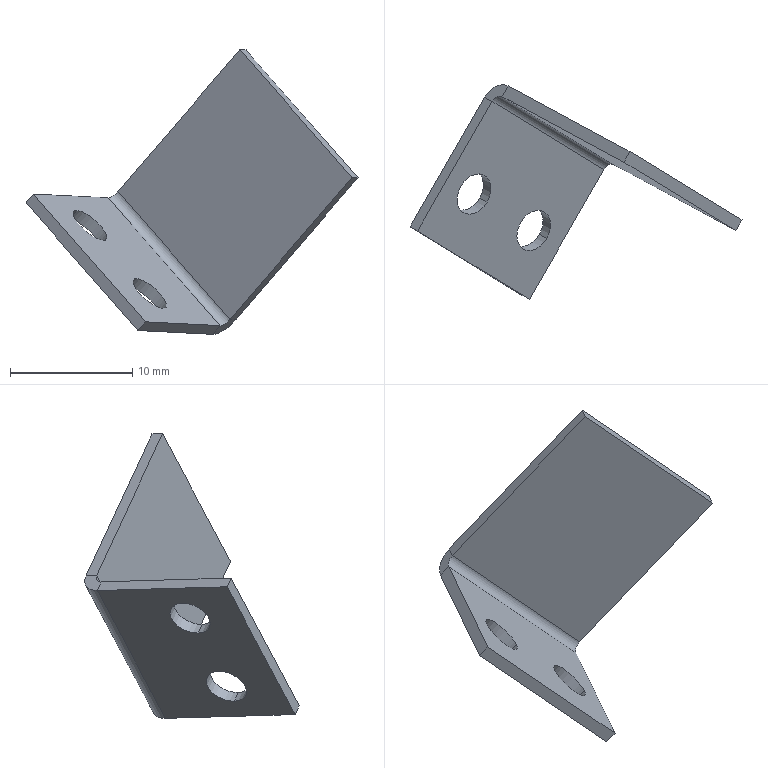Component | SolidWorks | ShadingPlateZ0-123-1 | 1 solid | 18 faces | box 27.21 x 17.57 x 23.33 mm | volume 438 mm3 | plane 12 | cylinder 6 | commonest cylinder face diameters 3.5 x4 3.473 x1 1.473 x1
STEP:
#1=COLOUR_RGB('',0.7922,0.8196,0.9333);
#2=FILL_AREA_STYLE_COLOUR('',#1);
#3=FILL_AREA_STYLE('',(#2));
#4=SURFACE_STYLE_FILL_AREA(#3);
#5=SURFACE_SIDE_STYLE('',(#4));
#6=SURFACE_STYLE_USAGE(.BOTH.,#5);
#7=PRESENTATION_STYLE_ASSIGNMENT((#6));
#8=CARTESIAN_POINT('',(2.839,-1.342,7.329));
#9=VERTEX_POINT('',#8);
#10=CARTESIAN_POINT('',(2.755,-1.29,7.425));
#11=VERTEX_POINT('',#10);
#12=CARTESIAN_POINT('',(2.797,-1.316,7.377));
#13=DIRECTION('',(0.6147,-0.3321,0.7154));
#14=DIRECTION('',(-0.6119,0.3716,0.6982));
#15=AXIS2_PLACEMENT_3D('',#12,#13,#14);
#16=CIRCLE('',#15,0.0689);
#17=EDGE_CURVE('',#9,#11,#16,.T.);
#18=ORIENTED_EDGE('',*,*,#17,.F.);
#19=CARTESIAN_POINT('',(2.864,-1.355,7.357));
#20=VERTEX_POINT('',#19);
#21=CARTESIAN_POINT('',(2.839,-1.342,7.329));
#22=DIRECTION('',(0.6147,-0.3321,0.7154));
#23=VECTOR('',#22,39.37);
#24=LINE('',#21,#23);
#25=EDGE_CURVE('',#9,#20,#24,.T.);
#26=ORIENTED_EDGE('',*,*,#25,.T.);
#27=CARTESIAN_POINT('',(2.779,-1.304,7.453));
#28=VERTEX_POINT('',#27);
#29=CARTESIAN_POINT('',(2.821,-1.329,7.405));
#30=DIRECTION('',(0.6147,-0.3321,0.7154));
#31=DIRECTION('',(-0.6119,0.3716,0.6982));
#32=AXIS2_PLACEMENT_3D('',#29,#30,#31);
#33=CIRCLE('',#32,0.0689);
#34=EDGE_CURVE('',#20,#28,#33,.T.);
#35=ORIENTED_EDGE('',*,*,#34,.T.);
#36=CARTESIAN_POINT('',(2.755,-1.29,7.425));
#37=DIRECTION('',(0.6147,-0.3321,0.7154));
#38=VECTOR('',#37,39.37);
#39=LINE('',#36,#38);
#40=EDGE_CURVE('',#11,#28,#39,.T.);
#41=ORIENTED_EDGE('',*,*,#40,.F.);
#42=EDGE_LOOP('',(#18,#26,#35,#41));
#43=FACE_OUTER_BOUND('',#42,.T.);
#44=CARTESIAN_POINT('',(2.797,-1.316,7.377));
#45=DIRECTION('',(0.6147,-0.3321,0.7154));
#46=DIRECTION('',(-0.6119,0.3716,0.6982));
#47=AXIS2_PLACEMENT_3D('',#44,#45,#46);
#48=CYLINDRICAL_SURFACE('',#47,0.0689);
#49=ADVANCED_FACE('',(#43),#48,.F.);
#50=CARTESIAN_POINT('',(3.032,-1.459,7.109));
#51=VERTEX_POINT('',#50);
#52=CARTESIAN_POINT('',(2.948,-1.407,7.205));
#53=VERTEX_POINT('',#52);
#54=CARTESIAN_POINT('',(2.99,-1.433,7.157));
#55=DIRECTION('',(0.6147,-0.3321,0.7154));
#56=DIRECTION('',(-0.6119,0.3716,0.6982));
#57=AXIS2_PLACEMENT_3D('',#54,#55,#56);
#58=CIRCLE('',#57,0.0689);
#59=EDGE_CURVE('',#51,#53,#58,.T.);
#60=ORIENTED_EDGE('',*,*,#59,.F.);
#61=CARTESIAN_POINT('',(3.056,-1.472,7.137));
#62=VERTEX_POINT('',#61);
#63=CARTESIAN_POINT('',(3.032,-1.459,7.109));
#64=DIRECTION('',(0.6147,-0.3321,0.7154));
#65=VECTOR('',#64,39.37);
#66=LINE('',#63,#65);
#67=EDGE_CURVE('',#51,#62,#66,.T.);
#68=ORIENTED_EDGE('',*,*,#67,.T.);
#69=CARTESIAN_POINT('',(2.972,-1.421,7.233));
#70=VERTEX_POINT('',#69);
#71=CARTESIAN_POINT('',(3.014,-1.446,7.185));
#72=DIRECTION('',(0.6147,-0.3321,0.7154));
#73=DIRECTION('',(-0.6119,0.3716,0.6982));
#74=AXIS2_PLACEMENT_3D('',#71,#72,#73);
#75=CIRCLE('',#74,0.0689);
#76=EDGE_CURVE('',#62,#70,#75,.T.);
#77=ORIENTED_EDGE('',*,*,#76,.T.);
#78=CARTESIAN_POINT('',(2.948,-1.407,7.205));
#79=DIRECTION('',(0.6147,-0.3321,0.7154));
#80=VECTOR('',#79,39.37);
#81=LINE('',#78,#80);
#82=EDGE_CURVE('',#53,#70,#81,.T.);
#83=ORIENTED_EDGE('',*,*,#82,.F.);
#84=EDGE_LOOP('',(#60,#68,#77,#83));
#85=FACE_OUTER_BOUND('',#84,.T.);
#86=CARTESIAN_POINT('',(2.99,-1.433,7.157));
#87=DIRECTION('',(0.6147,-0.3321,0.7154));
#88=DIRECTION('',(-0.6119,0.3716,0.6982));
#89=AXIS2_PLACEMENT_3D('',#86,#87,#88);
#90=CYLINDRICAL_SURFACE('',#89,0.0689);
#91=ADVANCED_FACE('',(#85),#90,.F.);
#92=CARTESIAN_POINT('',(2.879,-1.03,7.494));
#93=VERTEX_POINT('',#92);
#94=CARTESIAN_POINT('',(2.639,-1.449,7.506));
#95=VERTEX_POINT('',#94);
#96=CARTESIAN_POINT('',(2.639,-1.449,7.506));
#97=DIRECTION('',(-0.4977,-0.867,0.02519));
#98=VECTOR('',#97,39.37);
#99=LINE('',#96,#98);
#100=EDGE_CURVE('',#93,#95,#99,.T.);
#101=ORIENTED_EDGE('',*,*,#100,.F.);
#102=CARTESIAN_POINT('',(2.855,-1.017,7.466));
#103=VERTEX_POINT('',#102);
#104=CARTESIAN_POINT('',(2.879,-1.03,7.494));
#105=DIRECTION('',(-0.6147,0.3321,-0.7154));
#106=VECTOR('',#105,39.37);
#107=LINE('',#104,#106);
#108=EDGE_CURVE('',#93,#103,#107,.T.);
#109=ORIENTED_EDGE('',*,*,#108,.T.);
#110=CARTESIAN_POINT('',(2.615,-1.435,7.478));
#111=VERTEX_POINT('',#110);
#112=CARTESIAN_POINT('',(2.615,-1.435,7.478));
#113=DIRECTION('',(-0.4977,-0.867,0.02519));
#114=VECTOR('',#113,39.37);
#115=LINE('',#112,#114);
#116=EDGE_CURVE('',#103,#111,#115,.T.);
#117=ORIENTED_EDGE('',*,*,#116,.T.);
#118=CARTESIAN_POINT('',(2.615,-1.435,7.478));
#119=DIRECTION('',(0.6147,-0.3321,0.7154));
#120=VECTOR('',#119,39.37);
#121=LINE('',#118,#120);
#122=EDGE_CURVE('',#111,#95,#121,.T.);
#123=ORIENTED_EDGE('',*,*,#122,.T.);
#124=EDGE_LOOP('',(#101,#109,#117,#123));
#125=FACE_OUTER_BOUND('',#124,.T.);
#126=CARTESIAN_POINT('',(2.615,-1.435,7.478));
#127=DIRECTION('',(-0.6119,0.3716,0.6982));
#128=DIRECTION('',(-0.4977,-0.867,0.02519));
#129=AXIS2_PLACEMENT_3D('',#126,#127,#128);
#130=PLANE('',#129);
#131=ADVANCED_FACE('',(#125),#130,.T.);
#132=CARTESIAN_POINT('',(2.797,-1.316,7.377));
#133=DIRECTION('',(0.6147,-0.3321,0.7154));
#134=DIRECTION('',(-0.6119,0.3716,0.6982));
#135=AXIS2_PLACEMENT_3D('',#132,#133,#134);
#136=CIRCLE('',#135,0.0689);
#137=EDGE_CURVE('',#11,#9,#136,.T.);
#138=ORIENTED_EDGE('',*,*,#137,.T.);
#139=ORIENTED_EDGE('',*,*,#17,.T.);
#140=EDGE_LOOP('',(#138,#139));
#141=FACE_BOUND('',#140,.T.);
#142=CARTESIAN_POINT('',(2.99,-1.433,7.157));
#143=DIRECTION('',(0.6147,-0.3321,0.7154));
#144=DIRECTION('',(-0.6119,0.3716,0.6982));
#145=AXIS2_PLACEMENT_3D('',#142,#143,#144);
#146=CIRCLE('',#145,0.0689);
#147=EDGE_CURVE('',#53,#51,#146,.T.);
#148=ORIENTED_EDGE('',*,*,#147,.T.);
#149=ORIENTED_EDGE('',*,*,#59,.T.);
#150=EDGE_LOOP('',(#148,#149));
#151=FACE_BOUND('',#150,.T.);
#152=CARTESIAN_POINT('',(3.217,-1.236,7.054));
#153=VERTEX_POINT('',#152);
#154=CARTESIAN_POINT('',(2.855,-1.017,7.466));
#155=DIRECTION('',(0.6119,-0.3716,-0.6982));
#156=VECTOR('',#155,39.37);
#157=LINE('',#154,#156);
#158=EDGE_CURVE('',#103,#153,#157,.T.);
#159=ORIENTED_EDGE('',*,*,#158,.T.);
#160=CARTESIAN_POINT('',(2.976,-1.655,7.066));
#161=VERTEX_POINT('',#160);
#162=CARTESIAN_POINT('',(2.976,-1.655,7.066));
#163=DIRECTION('',(0.4977,0.867,-0.02519));
#164=VECTOR('',#163,39.37);
#165=LINE('',#162,#164);
#166=EDGE_CURVE('',#161,#153,#165,.T.);
#167=ORIENTED_EDGE('',*,*,#166,.F.);
#168=CARTESIAN_POINT('',(2.976,-1.655,7.066));
#169=DIRECTION('',(0.6119,-0.3716,-0.6982));
#170=VECTOR('',#169,39.37);
#171=LINE('',#168,#170);
#172=EDGE_CURVE('',#111,#161,#171,.T.);
#173=ORIENTED_EDGE('',*,*,#172,.F.);
#174=ORIENTED_EDGE('',*,*,#116,.F.);
#175=EDGE_LOOP('',(#159,#167,#173,#174));
#176=FACE_OUTER_BOUND('',#175,.T.);
#177=CARTESIAN_POINT('',(2.923,-1.323,7.265));
#178=DIRECTION('',(0.6147,-0.3321,0.7154));
#179=DIRECTION('',(-0.6119,0.3716,0.6982));
#180=AXIS2_PLACEMENT_3D('',#177,#178,#179);
#181=PLANE('',#180);
#182=ADVANCED_FACE('',(#141,#151,#176),#181,.F.);
#183=CARTESIAN_POINT('',(2.821,-1.329,7.405));
#184=DIRECTION('',(0.6147,-0.3321,0.7154));
#185=DIRECTION('',(-0.6119,0.3716,0.6982));
#186=AXIS2_PLACEMENT_3D('',#183,#184,#185);
#187=CIRCLE('',#186,0.0689);
#188=EDGE_CURVE('',#28,#20,#187,.T.);
#189=ORIENTED_EDGE('',*,*,#188,.F.);
#190=ORIENTED_EDGE('',*,*,#34,.F.);
#191=EDGE_LOOP('',(#189,#190));
#192=FACE_BOUND('',#191,.T.);
#193=CARTESIAN_POINT('',(3.014,-1.446,7.185));
#194=DIRECTION('',(0.6147,-0.3321,0.7154));
#195=DIRECTION('',(-0.6119,0.3716,0.6982));
#196=AXIS2_PLACEMENT_3D('',#193,#194,#195);
#197=CIRCLE('',#196,0.0689);
#198=EDGE_CURVE('',#70,#62,#197,.T.);
#199=ORIENTED_EDGE('',*,*,#198,.F.);
#200=ORIENTED_EDGE('',*,*,#76,.F.);
#201=EDGE_LOOP('',(#199,#200));
#202=FACE_BOUND('',#201,.T.);
#203=CARTESIAN_POINT('',(3.,-1.668,7.094));
#204=VERTEX_POINT('',#203);
#205=CARTESIAN_POINT('',(3.241,-1.249,7.082));
#206=VERTEX_POINT('',#205);
#207=CARTESIAN_POINT('',(3.,-1.668,7.094));
#208=DIRECTION('',(0.4977,0.867,-0.02519));
#209=VECTOR('',#208,39.37);
#210=LINE('',#207,#209);
#211=EDGE_CURVE('',#204,#206,#210,.T.);
#212=ORIENTED_EDGE('',*,*,#211,.T.);
#213=CARTESIAN_POINT('',(2.879,-1.03,7.494));
#214=DIRECTION('',(0.6119,-0.3716,-0.6982));
#215=VECTOR('',#214,39.37);
#216=LINE('',#213,#215);
#217=EDGE_CURVE('',#93,#206,#216,.T.);
#218=ORIENTED_EDGE('',*,*,#217,.F.);
#219=ORIENTED_EDGE('',*,*,#100,.T.);
#220=CARTESIAN_POINT('',(3.,-1.668,7.094));
#221=DIRECTION('',(0.6119,-0.3716,-0.6982));
#222=VECTOR('',#221,39.37);
#223=LINE('',#220,#222);
#224=EDGE_CURVE('',#95,#204,#223,.T.);
#225=ORIENTED_EDGE('',*,*,#224,.T.);
#226=EDGE_LOOP('',(#212,#218,#219,#225));
#227=FACE_OUTER_BOUND('',#226,.T.);
#228=CARTESIAN_POINT('',(2.947,-1.336,7.294));
#229=DIRECTION('',(0.6147,-0.3321,0.7154));
#230=DIRECTION('',(-0.6119,0.3716,0.6982));
#231=AXIS2_PLACEMENT_3D('',#228,#229,#230);
#232=PLANE('',#231);
#233=ADVANCED_FACE('',(#192,#202,#227),#232,.T.);
#234=CARTESIAN_POINT('',(3.241,-1.249,7.082));
#235=DIRECTION('',(-0.6147,0.3321,-0.7154));
#236=VECTOR('',#235,39.37);
#237=LINE('',#234,#236);
#238=EDGE_CURVE('',#206,#153,#237,.T.);
#239=ORIENTED_EDGE('',*,*,#238,.F.);
#240=ORIENTED_EDGE('',*,*,#211,.F.);
#241=CARTESIAN_POINT('',(2.976,-1.655,7.066));
#242=DIRECTION('',(0.6147,-0.3321,0.7154));
#243=VECTOR('',#242,39.37);
#244=LINE('',#241,#243);
#245=EDGE_CURVE('',#161,#204,#244,.T.);
#246=ORIENTED_EDGE('',*,*,#245,.F.);
#247=ORIENTED_EDGE('',*,*,#166,.T.);
#248=EDGE_LOOP('',(#239,#240,#246,#247));
#249=FACE_OUTER_BOUND('',#248,.T.);
#250=CARTESIAN_POINT('',(2.976,-1.655,7.066));
#251=DIRECTION('',(0.6119,-0.3716,-0.6982));
#252=DIRECTION('',(0.4977,0.867,-0.02519));
#253=AXIS2_PLACEMENT_3D('',#250,#251,#252);
#254=PLANE('',#253);
#255=ADVANCED_FACE('',(#249),#254,.T.);
#256=ORIENTED_EDGE('',*,*,#224,.F.);
#257=ORIENTED_EDGE('',*,*,#122,.F.);
#258=ORIENTED_EDGE('',*,*,#172,.T.);
#259=ORIENTED_EDGE('',*,*,#245,.T.);
#260=EDGE_LOOP('',(#256,#257,#258,#259));
#261=FACE_OUTER_BOUND('',#260,.T.);
#262=CARTESIAN_POINT('',(2.976,-1.655,7.066));
#263=DIRECTION('',(-0.4977,-0.867,0.02519));
#264=DIRECTION('',(0.6147,-0.3321,0.7154));
#265=AXIS2_PLACEMENT_3D('',#262,#263,#264);
#266=PLANE('',#265);
#267=ADVANCED_FACE('',(#261),#266,.T.);
#268=CARTESIAN_POINT('',(3.273,-1.234,7.102));
#269=VERTEX_POINT('',#268);
#270=CARTESIAN_POINT('',(3.293,-1.2,7.101));
#271=VERTEX_POINT('',#270);
#272=CARTESIAN_POINT('',(3.273,-1.234,7.102));
#273=DIRECTION('',(0.4977,0.867,-0.02519));
#274=VECTOR('',#273,39.37);
#275=LINE('',#272,#274);
#276=EDGE_CURVE('',#269,#271,#275,.T.);
#277=ORIENTED_EDGE('',*,*,#276,.F.);
#278=CARTESIAN_POINT('',(3.259,-1.259,7.102));
#279=DIRECTION('',(0.6119,-0.3716,-0.6982));
#280=DIRECTION('',(-0.6147,0.3321,-0.7154));
#281=AXIS2_PLACEMENT_3D('',#278,#279,#280);
#282=CIRCLE('',#281,0.029);
#283=EDGE_CURVE('',#206,#269,#282,.T.);
#284=ORIENTED_EDGE('',*,*,#283,.F.);
#285=ORIENTED_EDGE('',*,*,#238,.T.);
#286=CARTESIAN_POINT('',(3.259,-1.259,7.102));
#287=DIRECTION('',(0.6119,-0.3716,-0.6982));
#288=DIRECTION('',(-0.6147,0.3321,-0.7154));
#289=AXIS2_PLACEMENT_3D('',#286,#287,#288);
#290=CIRCLE('',#289,0.06837);
#291=EDGE_CURVE('',#153,#271,#290,.T.);
#292=ORIENTED_EDGE('',*,*,#291,.T.);
#293=EDGE_LOOP('',(#277,#284,#285,#292));
#294=FACE_OUTER_BOUND('',#293,.T.);
#295=CARTESIAN_POINT('',(3.259,-1.259,7.102));
#296=DIRECTION('',(0.6119,-0.3716,-0.6982));
#297=DIRECTION('',(0.6147,-0.3321,0.7154));
#298=AXIS2_PLACEMENT_3D('',#295,#296,#297);
#299=PLANE('',#298);
#300=ADVANCED_FACE('',(#294),#299,.T.);
#301=CARTESIAN_POINT('',(2.912,-1.014,7.514));
#302=VERTEX_POINT('',#301);
#303=CARTESIAN_POINT('',(2.897,-1.04,7.515));
#304=DIRECTION('',(-0.6119,0.3716,0.6982));
#305=DIRECTION('',(-0.6147,0.3321,-0.7154));
#306=AXIS2_PLACEMENT_3D('',#303,#304,#305);
#307=CIRCLE('',#306,0.029);
#308=EDGE_CURVE('',#302,#93,#307,.T.);
#309=ORIENTED_EDGE('',*,*,#308,.F.);
#310=CARTESIAN_POINT('',(2.931,-0.9803,7.513));
#311=VERTEX_POINT('',#310);
#312=CARTESIAN_POINT('',(2.912,-1.014,7.514));
#313=DIRECTION('',(0.4977,0.867,-0.02519));
#314=VECTOR('',#313,39.37);
#315=LINE('',#312,#314);
#316=EDGE_CURVE('',#302,#311,#315,.T.);
#317=ORIENTED_EDGE('',*,*,#316,.T.);
#318=CARTESIAN_POINT('',(2.897,-1.04,7.515));
#319=DIRECTION('',(-0.6119,0.3716,0.6982));
#320=DIRECTION('',(-0.6147,0.3321,-0.7154));
#321=AXIS2_PLACEMENT_3D('',#318,#319,#320);
#322=CIRCLE('',#321,0.06837);
#323=EDGE_CURVE('',#311,#103,#322,.T.);
#324=ORIENTED_EDGE('',*,*,#323,.T.);
#325=ORIENTED_EDGE('',*,*,#108,.F.);
#326=EDGE_LOOP('',(#309,#317,#324,#325));
#327=FACE_OUTER_BOUND('',#326,.T.);
#328=CARTESIAN_POINT('',(2.897,-1.04,7.515));
#329=DIRECTION('',(0.6119,-0.3716,-0.6982));
#330=DIRECTION('',(0.6147,-0.3321,0.7154));
#331=AXIS2_PLACEMENT_3D('',#328,#329,#330);
#332=PLANE('',#331);
#333=ADVANCED_FACE('',(#327),#332,.F.);
#334=ORIENTED_EDGE('',*,*,#158,.F.);
#335=ORIENTED_EDGE('',*,*,#323,.F.);
#336=CARTESIAN_POINT('',(3.112,-1.09,7.307));
#337=DIRECTION('',(0.6119,-0.3716,-0.6982));
#338=VECTOR('',#337,39.37);
#339=LINE('',#336,#338);
#340=EDGE_CURVE('',#311,#271,#339,.T.);
#341=ORIENTED_EDGE('',*,*,#340,.T.);
#342=ORIENTED_EDGE('',*,*,#291,.F.);
#343=EDGE_LOOP('',(#334,#335,#341,#342));
#344=FACE_OUTER_BOUND('',#343,.T.);
#345=CARTESIAN_POINT('',(2.897,-1.04,7.515));
#346=DIRECTION('',(-0.6119,0.3716,0.6982));
#347=DIRECTION('',(0.4977,0.867,-0.02519));
#348=AXIS2_PLACEMENT_3D('',#345,#346,#347);
#349=CYLINDRICAL_SURFACE('',#348,0.06837);
#350=ADVANCED_FACE('',(#344),#349,.T.);
#351=ORIENTED_EDGE('',*,*,#217,.T.);
#352=ORIENTED_EDGE('',*,*,#283,.T.);
#353=CARTESIAN_POINT('',(3.273,-1.234,7.102));
#354=DIRECTION('',(-0.6119,0.3716,0.6982));
#355=VECTOR('',#354,39.37);
#356=LINE('',#353,#355);
#357=EDGE_CURVE('',#269,#302,#356,.T.);
#358=ORIENTED_EDGE('',*,*,#357,.T.);
#359=ORIENTED_EDGE('',*,*,#308,.T.);
#360=EDGE_LOOP('',(#351,#352,#358,#359));
#361=FACE_OUTER_BOUND('',#360,.T.);
#362=CARTESIAN_POINT('',(2.897,-1.04,7.515));
#363=DIRECTION('',(-0.6119,0.3716,0.6982));
#364=DIRECTION('',(0.4977,0.867,-0.02519));
#365=AXIS2_PLACEMENT_3D('',#362,#363,#364);
#366=CYLINDRICAL_SURFACE('',#365,0.029);
#367=ADVANCED_FACE('',(#361),#366,.F.);
#368=ORIENTED_EDGE('',*,*,#276,.T.);
#369=CARTESIAN_POINT('',(3.686,-1.412,7.559));
#370=VERTEX_POINT('',#369);
#371=CARTESIAN_POINT('',(3.275,-1.19,7.08));
#372=DIRECTION('',(-0.6147,0.3321,-0.7154));
#373=VECTOR('',#372,39.37);
#374=LINE('',#371,#373);
#375=EDGE_CURVE('',#370,#271,#374,.T.);
#376=ORIENTED_EDGE('',*,*,#375,.F.);
#377=CARTESIAN_POINT('',(3.667,-1.447,7.56));
#378=VERTEX_POINT('',#377);
#379=CARTESIAN_POINT('',(3.686,-1.412,7.559));
#380=DIRECTION('',(-0.4977,-0.867,0.02519));
#381=VECTOR('',#380,39.37);
#382=LINE('',#379,#381);
#383=EDGE_CURVE('',#370,#378,#382,.T.);
#384=ORIENTED_EDGE('',*,*,#383,.T.);
#385=CARTESIAN_POINT('',(3.255,-1.224,7.081));
#386=DIRECTION('',(-0.6147,0.3321,-0.7154));
#387=VECTOR('',#386,39.37);
#388=LINE('',#385,#387);
#389=EDGE_CURVE('',#378,#269,#388,.T.);
#390=ORIENTED_EDGE('',*,*,#389,.T.);
#391=EDGE_LOOP('',(#368,#376,#384,#390));
#392=FACE_OUTER_BOUND('',#391,.T.);
#393=CARTESIAN_POINT('',(3.275,-1.19,7.08));
#394=DIRECTION('',(-0.6119,0.3716,0.6982));
#395=DIRECTION('',(-0.6147,0.3321,-0.7154));
#396=AXIS2_PLACEMENT_3D('',#393,#394,#395);
#397=PLANE('',#396);
#398=ADVANCED_FACE('',(#392),#397,.F.);
#399=ORIENTED_EDGE('',*,*,#316,.F.);
#400=CARTESIAN_POINT('',(3.305,-1.227,7.972));
#401=VERTEX_POINT('',#400);
#402=CARTESIAN_POINT('',(3.305,-1.227,7.972));
#403=DIRECTION('',(0.6147,-0.3321,0.7154));
#404=VECTOR('',#403,39.37);
#405=LINE('',#402,#404);
#406=EDGE_CURVE('',#302,#401,#405,.T.);
#407=ORIENTED_EDGE('',*,*,#406,.T.);
#408=CARTESIAN_POINT('',(3.325,-1.193,7.971));
#409=VERTEX_POINT('',#408);
#410=CARTESIAN_POINT('',(3.325,-1.193,7.971));
#411=DIRECTION('',(-0.4977,-0.867,0.02519));
#412=VECTOR('',#411,39.37);
#413=LINE('',#410,#412);
#414=EDGE_CURVE('',#409,#401,#413,.T.);
#415=ORIENTED_EDGE('',*,*,#414,.F.);
#416=CARTESIAN_POINT('',(3.325,-1.193,7.971));
#417=DIRECTION('',(0.6147,-0.3321,0.7154));
#418=VECTOR('',#417,39.37);
#419=LINE('',#416,#418);
#420=EDGE_CURVE('',#311,#409,#419,.T.);
#421=ORIENTED_EDGE('',*,*,#420,.F.);
#422=EDGE_LOOP('',(#399,#407,#415,#421));
#423=FACE_OUTER_BOUND('',#422,.T.);
#424=CARTESIAN_POINT('',(3.325,-1.193,7.971));
#425=DIRECTION('',(0.6119,-0.3716,-0.6982));
#426=DIRECTION('',(0.6147,-0.3321,0.7154));
#427=AXIS2_PLACEMENT_3D('',#424,#425,#426);
#428=PLANE('',#427);
#429=ADVANCED_FACE('',(#423),#428,.F.);
#430=ORIENTED_EDGE('',*,*,#340,.F.);
#431=ORIENTED_EDGE('',*,*,#420,.T.);
#432=CARTESIAN_POINT('',(3.686,-1.412,7.559));
#433=DIRECTION('',(0.6119,-0.3716,-0.6982));
#434=VECTOR('',#433,39.37);
#435=LINE('',#432,#434);
#436=EDGE_CURVE('',#409,#370,#435,.T.);
#437=ORIENTED_EDGE('',*,*,#436,.T.);
#438=ORIENTED_EDGE('',*,*,#375,.T.);
#439=EDGE_LOOP('',(#430,#431,#437,#438));
#440=FACE_OUTER_BOUND('',#439,.T.);
#441=CARTESIAN_POINT('',(3.094,-1.08,7.286));
#442=DIRECTION('',(-0.4977,-0.867,0.02519));
#443=DIRECTION('',(0.6147,-0.3321,0.7154));
#444=AXIS2_PLACEMENT_3D('',#441,#442,#443);
#445=PLANE('',#444);
#446=ADVANCED_FACE('',(#440),#445,.F.);
#447=ORIENTED_EDGE('',*,*,#406,.F.);
#448=ORIENTED_EDGE('',*,*,#357,.F.);
#449=ORIENTED_EDGE('',*,*,#389,.F.);
#450=CARTESIAN_POINT('',(3.667,-1.447,7.56));
#451=DIRECTION('',(0.6119,-0.3716,-0.6982));
#452=VECTOR('',#451,39.37);
#453=LINE('',#450,#452);
#454=EDGE_CURVE('',#401,#378,#453,.T.);
#455=ORIENTED_EDGE('',*,*,#454,.F.);
#456=EDGE_LOOP('',(#447,#448,#449,#455));
#457=FACE_OUTER_BOUND('',#456,.T.);
#458=CARTESIAN_POINT('',(3.075,-1.115,7.287));
#459=DIRECTION('',(-0.4977,-0.867,0.02519));
#460=DIRECTION('',(0.6147,-0.3321,0.7154));
#461=AXIS2_PLACEMENT_3D('',#458,#459,#460);
#462=PLANE('',#461);
#463=ADVANCED_FACE('',(#457),#462,.T.);
#464=ORIENTED_EDGE('',*,*,#454,.T.);
#465=ORIENTED_EDGE('',*,*,#383,.F.);
#466=ORIENTED_EDGE('',*,*,#436,.F.);
#467=ORIENTED_EDGE('',*,*,#414,.T.);
#468=EDGE_LOOP('',(#464,#465,#466,#467));
#469=FACE_OUTER_BOUND('',#468,.T.);
#470=CARTESIAN_POINT('',(3.686,-1.412,7.559));
#471=DIRECTION('',(-0.6147,0.3321,-0.7154));
#472=DIRECTION('',(-0.4977,-0.867,0.02519));
#473=AXIS2_PLACEMENT_3D('',#470,#471,#472);
#474=PLANE('',#473);
#475=ADVANCED_FACE('',(#469),#474,.F.);
#476=ORIENTED_EDGE('',*,*,#67,.F.);
#477=ORIENTED_EDGE('',*,*,#147,.F.);
#478=ORIENTED_EDGE('',*,*,#82,.T.);
#479=ORIENTED_EDGE('',*,*,#198,.T.);
#480=EDGE_LOOP('',(#476,#477,#478,#479));
#481=FACE_OUTER_BOUND('',#480,.T.);
#482=CARTESIAN_POINT('',(2.99,-1.433,7.157));
#483=DIRECTION('',(0.6147,-0.3321,0.7154));
#484=DIRECTION('',(-0.6119,0.3716,0.6982));
#485=AXIS2_PLACEMENT_3D('',#482,#483,#484);
#486=CYLINDRICAL_SURFACE('',#485,0.0689);
#487=ADVANCED_FACE('',(#481),#486,.F.);
#488=ORIENTED_EDGE('',*,*,#25,.F.);
#489=ORIENTED_EDGE('',*,*,#137,.F.);
#490=ORIENTED_EDGE('',*,*,#40,.T.);
#491=ORIENTED_EDGE('',*,*,#188,.T.);
#492=EDGE_LOOP('',(#488,#489,#490,#491));
#493=FACE_OUTER_BOUND('',#492,.T.);
#494=CARTESIAN_POINT('',(2.797,-1.316,7.377));
#495=DIRECTION('',(0.6147,-0.3321,0.7154));
#496=DIRECTION('',(-0.6119,0.3716,0.6982));
#497=AXIS2_PLACEMENT_3D('',#494,#495,#496);
#498=CYLINDRICAL_SURFACE('',#497,0.0689);
#499=ADVANCED_FACE('',(#493),#498,.F.);
#500=CLOSED_SHELL('',(#49,#91,#131,#182,#233,#255,#267,#300,#333,#350,#367,#398,#429,#446,#463,#475,#487,#499));
#501=MANIFOLD_SOLID_BREP('',#500);
#502=STYLED_ITEM('',(#7),#501);
#503=PRESENTATION_LAYER_ASSIGNMENT('','',(#502));
#504=CARTESIAN_POINT('',(0.,0.,0.));
#505=DIRECTION('',(0.,0.,1.));
#506=DIRECTION('',(1.,0.,0.));
#507=AXIS2_PLACEMENT_3D('',#504,#505,#506);
#508=(LENGTH_UNIT()NAMED_UNIT(*)SI_UNIT($,.METRE.));
#509=LENGTH_MEASURE_WITH_UNIT(LENGTH_MEASURE(0.0254),#508);
#510=DIMENSIONAL_EXPONENTS(1.,0.,0.,0.,0.,0.,0.);
#511=(CONVERSION_BASED_UNIT('',#509)LENGTH_UNIT()NAMED_UNIT(#510));
#512=UNCERTAINTY_MEASURE_WITH_UNIT(LENGTH_MEASURE(0.00001),#511,'','');
#513=(NAMED_UNIT(*)PLANE_ANGLE_UNIT()SI_UNIT($,.RADIAN.));
#514=(NAMED_UNIT(*)SI_UNIT($,.STERADIAN.)SOLID_ANGLE_UNIT());
#515=(GEOMETRIC_REPRESENTATION_CONTEXT(3)GLOBAL_UNCERTAINTY_ASSIGNED_CONTEXT((#512))GLOBAL_UNIT_ASSIGNED_CONTEXT((#511,#513,#514))REPRESENTATION_CONTEXT('',''));
#516=ADVANCED_BREP_SHAPE_REPRESENTATION('',(#501,#507),#515);
#517=(LENGTH_UNIT()NAMED_UNIT(*)SI_UNIT($,.METRE.));
#518=LENGTH_MEASURE_WITH_UNIT(LENGTH_MEASURE(0.0254),#517);
#519=DIMENSIONAL_EXPONENTS(1.,0.,0.,0.,0.,0.,0.);
#520=(CONVERSION_BASED_UNIT('',#518)LENGTH_UNIT()NAMED_UNIT(#519));
#521=UNCERTAINTY_MEASURE_WITH_UNIT(LENGTH_MEASURE(0.00001),#520,'','');
#522=(NAMED_UNIT(*)PLANE_ANGLE_UNIT()SI_UNIT($,.RADIAN.));
#523=(NAMED_UNIT(*)SI_UNIT($,.STERADIAN.)SOLID_ANGLE_UNIT());
#524=(GEOMETRIC_REPRESENTATION_CONTEXT(3)GLOBAL_UNCERTAINTY_ASSIGNED_CONTEXT((#521))GLOBAL_UNIT_ASSIGNED_CONTEXT((#520,#522,#523))REPRESENTATION_CONTEXT('',''));
#525=MECHANICAL_DESIGN_GEOMETRIC_PRESENTATION_REPRESENTATION('',(#502),#524);